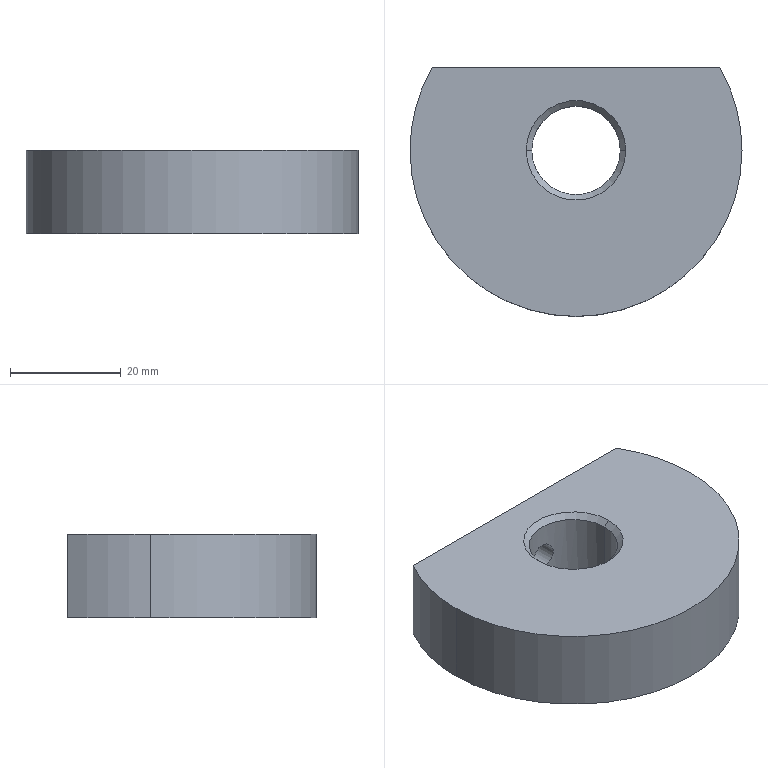Component | SolidWorks | YC1-250-09SecondDropAssembly-1_YC1-25-09-02Cam-1 | 1 solid | 14 faces | box 60 x 45 x 15 mm | volume 30912 mm3 | cylinder 7 | cone 4 | plane 3 | commonest cylinder face diameters 60 x3 5 x2 16 x2 | material Plain Carbon Steel
STEP:
#1=COLOUR_RGB('',0.7922,0.8196,0.9333);
#2=FILL_AREA_STYLE_COLOUR('',#1);
#3=FILL_AREA_STYLE('',(#2));
#4=SURFACE_STYLE_FILL_AREA(#3);
#5=SURFACE_SIDE_STYLE('',(#4));
#6=SURFACE_STYLE_USAGE(.BOTH.,#5);
#7=PRESENTATION_STYLE_ASSIGNMENT((#6));
#8=CARTESIAN_POINT('',(1.023,132.283,-41.024));
#9=VERTEX_POINT('',#8);
#10=CARTESIAN_POINT('',(1.181,131.693,-41.024));
#11=VERTEX_POINT('',#10);
#12=CARTESIAN_POINT('',(0.,131.693,-41.024));
#13=DIRECTION('',(0.,0.,-1.));
#14=DIRECTION('',(-1.,0.,0.));
#15=AXIS2_PLACEMENT_3D('',#12,#13,#14);
#16=CIRCLE('',#15,1.181);
#17=EDGE_CURVE('',#9,#11,#16,.T.);
#18=ORIENTED_EDGE('',*,*,#17,.T.);
#19=CARTESIAN_POINT('',(1.181,131.693,-41.614));
#20=VERTEX_POINT('',#19);
#21=CARTESIAN_POINT('',(1.181,131.693,-41.024));
#22=DIRECTION('',(0.,0.,-1.));
#23=VECTOR('',#22,39.37);
#24=LINE('',#21,#23);
#25=EDGE_CURVE('',#11,#20,#24,.T.);
#26=ORIENTED_EDGE('',*,*,#25,.T.);
#27=CARTESIAN_POINT('',(1.023,132.283,-41.614));
#28=VERTEX_POINT('',#27);
#29=CARTESIAN_POINT('',(0.,131.693,-41.614));
#30=DIRECTION('',(0.,0.,1.));
#31=DIRECTION('',(-1.,-0.,0.));
#32=AXIS2_PLACEMENT_3D('',#29,#30,#31);
#33=CIRCLE('',#32,1.181);
#34=EDGE_CURVE('',#20,#28,#33,.T.);
#35=ORIENTED_EDGE('',*,*,#34,.T.);
#36=CARTESIAN_POINT('',(1.023,132.283,-41.024));
#37=DIRECTION('',(0.,0.,1.));
#38=VECTOR('',#37,39.37);
#39=LINE('',#36,#38);
#40=EDGE_CURVE('',#28,#9,#39,.T.);
#41=ORIENTED_EDGE('',*,*,#40,.T.);
#42=EDGE_LOOP('',(#18,#26,#35,#41));
#43=FACE_OUTER_BOUND('',#42,.T.);
#44=CARTESIAN_POINT('',(0.,131.693,-41.024));
#45=DIRECTION('',(0.,0.,-1.));
#46=DIRECTION('',(-1.,0.,0.));
#47=AXIS2_PLACEMENT_3D('',#44,#45,#46);
#48=CYLINDRICAL_SURFACE('',#47,1.181);
#49=ADVANCED_FACE('',(#43),#48,.T.);
#50=ORIENTED_EDGE('',*,*,#25,.F.);
#51=CARTESIAN_POINT('',(-1.181,131.693,-41.024));
#52=VERTEX_POINT('',#51);
#53=CARTESIAN_POINT('',(0.,131.693,-41.024));
#54=DIRECTION('',(0.,0.,-1.));
#55=DIRECTION('',(-1.,0.,0.));
#56=AXIS2_PLACEMENT_3D('',#53,#54,#55);
#57=CIRCLE('',#56,1.181);
#58=EDGE_CURVE('',#11,#52,#57,.T.);
#59=ORIENTED_EDGE('',*,*,#58,.T.);
#60=CARTESIAN_POINT('',(-1.181,131.693,-41.614));
#61=VERTEX_POINT('',#60);
#62=CARTESIAN_POINT('',(-1.181,131.693,-41.024));
#63=DIRECTION('',(0.,0.,-1.));
#64=VECTOR('',#63,39.37);
#65=LINE('',#62,#64);
#66=EDGE_CURVE('',#52,#61,#65,.T.);
#67=ORIENTED_EDGE('',*,*,#66,.T.);
#68=CARTESIAN_POINT('',(0.,131.693,-41.614));
#69=DIRECTION('',(0.,0.,1.));
#70=DIRECTION('',(-1.,0.,0.));
#71=AXIS2_PLACEMENT_3D('',#68,#69,#70);
#72=CIRCLE('',#71,1.181);
#73=EDGE_CURVE('',#61,#20,#72,.T.);
#74=ORIENTED_EDGE('',*,*,#73,.T.);
#75=EDGE_LOOP('',(#50,#59,#67,#74));
#76=FACE_OUTER_BOUND('',#75,.T.);
#77=CARTESIAN_POINT('',(0.,131.693,-41.024));
#78=DIRECTION('',(0.,0.,-1.));
#79=DIRECTION('',(-1.,0.,0.));
#80=AXIS2_PLACEMENT_3D('',#77,#78,#79);
#81=CYLINDRICAL_SURFACE('',#80,1.181);
#82=ADVANCED_FACE('',(#76),#81,.T.);
#83=CARTESIAN_POINT('',(0.,131.378,-41.575));
#84=VERTEX_POINT('',#83);
#85=CARTESIAN_POINT('',(-0.315,131.693,-41.575));
#86=VERTEX_POINT('',#85);
#87=CARTESIAN_POINT('',(0.,131.693,-41.575));
#88=DIRECTION('',(0.,0.,-1.));
#89=DIRECTION('',(-1.,0.,0.));
#90=AXIS2_PLACEMENT_3D('',#87,#88,#89);
#91=CIRCLE('',#90,0.315);
#92=EDGE_CURVE('',#84,#86,#91,.T.);
#93=ORIENTED_EDGE('',*,*,#92,.F.);
#94=CARTESIAN_POINT('',(0.,131.339,-41.614));
#95=VERTEX_POINT('',#94);
#96=CARTESIAN_POINT('',(0.,131.339,-41.614));
#97=DIRECTION('',(0.,-0.7071,-0.7071));
#98=VECTOR('',#97,39.37);
#99=LINE('',#96,#98);
#100=EDGE_CURVE('',#84,#95,#99,.T.);
#101=ORIENTED_EDGE('',*,*,#100,.T.);
#102=CARTESIAN_POINT('',(0.,132.047,-41.614));
#103=VERTEX_POINT('',#102);
#104=CARTESIAN_POINT('',(0.,131.693,-41.614));
#105=DIRECTION('',(0.,0.,-1.));
#106=DIRECTION('',(0.,1.,0.));
#107=AXIS2_PLACEMENT_3D('',#104,#105,#106);
#108=CIRCLE('',#107,0.3543);
#109=EDGE_CURVE('',#95,#103,#108,.T.);
#110=ORIENTED_EDGE('',*,*,#109,.T.);
#111=CARTESIAN_POINT('',(0.,132.008,-41.575));
#112=VERTEX_POINT('',#111);
#113=CARTESIAN_POINT('',(0.,132.047,-41.614));
#114=DIRECTION('',(0.,0.7071,-0.7071));
#115=VECTOR('',#114,39.37);
#116=LINE('',#113,#115);
#117=EDGE_CURVE('',#112,#103,#116,.T.);
#118=ORIENTED_EDGE('',*,*,#117,.F.);
#119=CARTESIAN_POINT('',(0.,131.693,-41.575));
#120=DIRECTION('',(0.,0.,-1.));
#121=DIRECTION('',(-1.,0.,0.));
#122=AXIS2_PLACEMENT_3D('',#119,#120,#121);
#123=CIRCLE('',#122,0.315);
#124=EDGE_CURVE('',#86,#112,#123,.T.);
#125=ORIENTED_EDGE('',*,*,#124,.F.);
#126=EDGE_LOOP('',(#93,#101,#110,#118,#125));
#127=FACE_OUTER_BOUND('',#126,.T.);
#128=CARTESIAN_POINT('',(0.,131.693,-41.614));
#129=DIRECTION('',(0.,0.,-1.));
#130=DIRECTION('',(0.,1.,0.));
#131=AXIS2_PLACEMENT_3D('',#128,#129,#130);
#132=CONICAL_SURFACE('',#131,0.3543,0.7854);
#133=ADVANCED_FACE('',(#127),#132,.F.);
#134=CARTESIAN_POINT('',(0.,132.008,-41.417));
#135=VERTEX_POINT('',#134);
#136=CARTESIAN_POINT('',(0.,132.008,-41.22));
#137=VERTEX_POINT('',#136);
#138=CARTESIAN_POINT('',(0.,132.008,-41.417));
#139=CARTESIAN_POINT('',(-0.006545,132.008,-41.417));
#140=CARTESIAN_POINT('',(-0.01297,132.008,-41.417));
#141=CARTESIAN_POINT('',(-0.02561,132.007,-41.414));
#142=CARTESIAN_POINT('',(-0.03188,132.006,-41.412));
#143=CARTESIAN_POINT('',(-0.04378,132.005,-41.407));
#144=CARTESIAN_POINT('',(-0.04942,132.004,-41.404));
#145=CARTESIAN_POINT('',(-0.06008,132.002,-41.397));
#146=CARTESIAN_POINT('',(-0.0651,132.001,-41.393));
#147=CARTESIAN_POINT('',(-0.07862,131.998,-41.379));
#148=CARTESIAN_POINT('',(-0.08593,131.996,-41.369));
#149=CARTESIAN_POINT('',(-0.09332,131.994,-41.351));
#150=CARTESIAN_POINT('',(-0.09523,131.993,-41.345));
#151=CARTESIAN_POINT('',(-0.09778,131.992,-41.332));
#152=CARTESIAN_POINT('',(-0.09842,131.992,-41.325));
#153=CARTESIAN_POINT('',(-0.09843,131.992,-41.313));
#154=CARTESIAN_POINT('',(-0.09779,131.992,-41.306));
#155=CARTESIAN_POINT('',(-0.09526,131.993,-41.293));
#156=CARTESIAN_POINT('',(-0.09339,131.994,-41.287));
#157=CARTESIAN_POINT('',(-0.08843,131.995,-41.275));
#158=CARTESIAN_POINT('',(-0.08537,131.996,-41.27));
#159=CARTESIAN_POINT('',(-0.07827,131.998,-41.259));
#160=CARTESIAN_POINT('',(-0.07417,131.999,-41.254));
#161=CARTESIAN_POINT('',(-0.0651,132.001,-41.245));
#162=CARTESIAN_POINT('',(-0.06018,132.002,-41.241));
#163=CARTESIAN_POINT('',(-0.04955,132.004,-41.234));
#164=CARTESIAN_POINT('',(-0.04379,132.005,-41.231));
#165=CARTESIAN_POINT('',(-0.03194,132.006,-41.226));
#166=CARTESIAN_POINT('',(-0.0258,132.007,-41.224));
#167=CARTESIAN_POINT('',(-0.01309,132.008,-41.221));
#168=CARTESIAN_POINT('',(-0.006544,132.008,-41.22));
#169=CARTESIAN_POINT('',(0.,132.008,-41.22));
#170=B_SPLINE_CURVE_WITH_KNOTS('',3,(#138,#139,#140,#141,#142,#143,#144,#145,#146,#147,#148,#149,#150,#151,#152,#153,#154,#155,#156,#157,#158,#159,#160,#161,#162,#163,#164,#165,#166,#167,#168,#169),.UNSPECIFIED.,.F.,.F.,(4,2,2,2,2,2,2,2,2,2,2,2,2,2,2,4),(0.007863,0.008354,0.008846,0.009337,0.009828,0.01081,0.0113,0.01179,0.01229,0.01278,0.01327,0.01376,0.01425,0.01474,0.01523,0.01573),.UNSPECIFIED.);
#171=EDGE_CURVE('',#135,#137,#170,.T.);
#172=ORIENTED_EDGE('',*,*,#171,.F.);
#173=CARTESIAN_POINT('',(0.,132.283,-41.417));
#174=VERTEX_POINT('',#173);
#175=CARTESIAN_POINT('',(0.,132.283,-41.417));
#176=DIRECTION('',(0.,1.,0.));
#177=VECTOR('',#176,39.37);
#178=LINE('',#175,#177);
#179=EDGE_CURVE('',#135,#174,#178,.T.);
#180=ORIENTED_EDGE('',*,*,#179,.T.);
#181=CARTESIAN_POINT('',(0.,132.283,-41.22));
#182=VERTEX_POINT('',#181);
#183=CARTESIAN_POINT('',(0.,132.283,-41.319));
#184=DIRECTION('',(0.,1.,0.));
#185=DIRECTION('',(0.,0.,1.));
#186=AXIS2_PLACEMENT_3D('',#183,#184,#185);
#187=CIRCLE('',#186,0.09843);
#188=EDGE_CURVE('',#174,#182,#187,.T.);
#189=ORIENTED_EDGE('',*,*,#188,.T.);
#190=CARTESIAN_POINT('',(0.,132.283,-41.22));
#191=DIRECTION('',(0.,1.,0.));
#192=VECTOR('',#191,39.37);
#193=LINE('',#190,#192);
#194=EDGE_CURVE('',#137,#182,#193,.T.);
#195=ORIENTED_EDGE('',*,*,#194,.F.);
#196=EDGE_LOOP('',(#172,#180,#189,#195));
#197=FACE_OUTER_BOUND('',#196,.T.);
#198=CARTESIAN_POINT('',(0.,132.283,-41.319));
#199=DIRECTION('',(0.,1.,0.));
#200=DIRECTION('',(0.,0.,1.));
#201=AXIS2_PLACEMENT_3D('',#198,#199,#200);
#202=CYLINDRICAL_SURFACE('',#201,0.09843);
#203=ADVANCED_FACE('',(#197),#202,.F.);
#204=CARTESIAN_POINT('',(0.315,131.693,-41.063));
#205=VERTEX_POINT('',#204);
#206=CARTESIAN_POINT('',(-0.315,131.693,-41.063));
#207=VERTEX_POINT('',#206);
#208=CARTESIAN_POINT('',(0.,131.693,-41.063));
#209=DIRECTION('',(0.,0.,-1.));
#210=DIRECTION('',(-1.,0.,0.));
#211=AXIS2_PLACEMENT_3D('',#208,#209,#210);
#212=CIRCLE('',#211,0.315);
#213=EDGE_CURVE('',#205,#207,#212,.T.);
#214=ORIENTED_EDGE('',*,*,#213,.F.);
#215=CARTESIAN_POINT('',(0.315,131.693,-41.575));
#216=VERTEX_POINT('',#215);
#217=CARTESIAN_POINT('',(0.315,131.693,-41.024));
#218=DIRECTION('',(0.,0.,-1.));
#219=VECTOR('',#218,39.37);
#220=LINE('',#217,#219);
#221=EDGE_CURVE('',#205,#216,#220,.T.);
#222=ORIENTED_EDGE('',*,*,#221,.T.);
#223=CARTESIAN_POINT('',(0.,131.693,-41.575));
#224=DIRECTION('',(0.,0.,-1.));
#225=DIRECTION('',(-1.,0.,0.));
#226=AXIS2_PLACEMENT_3D('',#223,#224,#225);
#227=CIRCLE('',#226,0.315);
#228=EDGE_CURVE('',#216,#84,#227,.T.);
#229=ORIENTED_EDGE('',*,*,#228,.T.);
#230=ORIENTED_EDGE('',*,*,#92,.T.);
#231=CARTESIAN_POINT('',(-0.315,131.693,-41.024));
#232=DIRECTION('',(0.,0.,-1.));
#233=VECTOR('',#232,39.37);
#234=LINE('',#231,#233);
#235=EDGE_CURVE('',#207,#86,#234,.T.);
#236=ORIENTED_EDGE('',*,*,#235,.F.);
#237=EDGE_LOOP('',(#214,#222,#229,#230,#236));
#238=FACE_OUTER_BOUND('',#237,.T.);
#239=CARTESIAN_POINT('',(0.,131.693,-41.024));
#240=DIRECTION('',(0.,0.,-1.));
#241=DIRECTION('',(-1.,0.,0.));
#242=AXIS2_PLACEMENT_3D('',#239,#240,#241);
#243=CYLINDRICAL_SURFACE('',#242,0.315);
#244=ADVANCED_FACE('',(#238),#243,.F.);
#245=ORIENTED_EDGE('',*,*,#213,.T.);
#246=CARTESIAN_POINT('',(-0.3543,131.693,-41.024));
#247=VERTEX_POINT('',#246);
#248=CARTESIAN_POINT('',(-0.3543,131.693,-41.024));
#249=DIRECTION('',(-0.7071,0.,0.7071));
#250=VECTOR('',#249,39.37);
#251=LINE('',#248,#250);
#252=EDGE_CURVE('',#207,#247,#251,.T.);
#253=ORIENTED_EDGE('',*,*,#252,.T.);
#254=CARTESIAN_POINT('',(0.3543,131.693,-41.024));
#255=VERTEX_POINT('',#254);
#256=CARTESIAN_POINT('',(0.,131.693,-41.024));
#257=DIRECTION('',(0.,0.,-1.));
#258=DIRECTION('',(1.,0.,0.));
#259=AXIS2_PLACEMENT_3D('',#256,#257,#258);
#260=CIRCLE('',#259,0.3543);
#261=EDGE_CURVE('',#255,#247,#260,.T.);
#262=ORIENTED_EDGE('',*,*,#261,.F.);
#263=CARTESIAN_POINT('',(0.3543,131.693,-41.024));
#264=DIRECTION('',(0.7071,0.,0.7071));
#265=VECTOR('',#264,39.37);
#266=LINE('',#263,#265);
#267=EDGE_CURVE('',#205,#255,#266,.T.);
#268=ORIENTED_EDGE('',*,*,#267,.F.);
#269=EDGE_LOOP('',(#245,#253,#262,#268));
#270=FACE_OUTER_BOUND('',#269,.T.);
#271=CARTESIAN_POINT('',(0.,131.693,-41.024));
#272=DIRECTION('',(0.,0.,1.));
#273=DIRECTION('',(1.,0.,0.));
#274=AXIS2_PLACEMENT_3D('',#271,#272,#273);
#275=CONICAL_SURFACE('',#274,0.3543,0.7854);
#276=ADVANCED_FACE('',(#270),#275,.F.);
#277=CARTESIAN_POINT('',(-1.023,132.283,-41.614));
#278=VERTEX_POINT('',#277);
#279=CARTESIAN_POINT('',(0.,132.283,-41.614));
#280=DIRECTION('',(-1.,0.,0.));
#281=VECTOR('',#280,39.37);
#282=LINE('',#279,#281);
#283=EDGE_CURVE('',#28,#278,#282,.T.);
#284=ORIENTED_EDGE('',*,*,#283,.F.);
#285=ORIENTED_EDGE('',*,*,#34,.F.);
#286=ORIENTED_EDGE('',*,*,#73,.F.);
#287=CARTESIAN_POINT('',(0.,131.693,-41.614));
#288=DIRECTION('',(0.,0.,1.));
#289=DIRECTION('',(-1.,-0.,0.));
#290=AXIS2_PLACEMENT_3D('',#287,#288,#289);
#291=CIRCLE('',#290,1.181);
#292=EDGE_CURVE('',#278,#61,#291,.T.);
#293=ORIENTED_EDGE('',*,*,#292,.F.);
#294=EDGE_LOOP('',(#284,#285,#286,#293));
#295=FACE_OUTER_BOUND('',#294,.T.);
#296=CARTESIAN_POINT('',(0.,131.693,-41.614));
#297=DIRECTION('',(0.,0.,-1.));
#298=DIRECTION('',(0.,1.,0.));
#299=AXIS2_PLACEMENT_3D('',#296,#297,#298);
#300=CIRCLE('',#299,0.3543);
#301=EDGE_CURVE('',#103,#95,#300,.T.);
#302=ORIENTED_EDGE('',*,*,#301,.F.);
#303=ORIENTED_EDGE('',*,*,#109,.F.);
#304=EDGE_LOOP('',(#302,#303));
#305=FACE_BOUND('',#304,.T.);
#306=CARTESIAN_POINT('',(0.,131.693,-41.614));
#307=DIRECTION('',(0.,0.,1.));
#308=DIRECTION('',(1.,0.,0.));
#309=AXIS2_PLACEMENT_3D('',#306,#307,#308);
#310=PLANE('',#309);
#311=ADVANCED_FACE('',(#295,#305),#310,.F.);
#312=ORIENTED_EDGE('',*,*,#66,.F.);
#313=CARTESIAN_POINT('',(-1.023,132.283,-41.024));
#314=VERTEX_POINT('',#313);
#315=CARTESIAN_POINT('',(0.,131.693,-41.024));
#316=DIRECTION('',(0.,0.,-1.));
#317=DIRECTION('',(-1.,0.,0.));
#318=AXIS2_PLACEMENT_3D('',#315,#316,#317);
#319=CIRCLE('',#318,1.181);
#320=EDGE_CURVE('',#52,#314,#319,.T.);
#321=ORIENTED_EDGE('',*,*,#320,.T.);
#322=CARTESIAN_POINT('',(-1.023,132.283,-41.024));
#323=DIRECTION('',(0.,0.,-1.));
#324=VECTOR('',#323,39.37);
#325=LINE('',#322,#324);
#326=EDGE_CURVE('',#314,#278,#325,.T.);
#327=ORIENTED_EDGE('',*,*,#326,.T.);
#328=ORIENTED_EDGE('',*,*,#292,.T.);
#329=EDGE_LOOP('',(#312,#321,#327,#328));
#330=FACE_OUTER_BOUND('',#329,.T.);
#331=CARTESIAN_POINT('',(0.,131.693,-41.024));
#332=DIRECTION('',(0.,0.,-1.));
#333=DIRECTION('',(-1.,0.,0.));
#334=AXIS2_PLACEMENT_3D('',#331,#332,#333);
#335=CYLINDRICAL_SURFACE('',#334,1.181);
#336=ADVANCED_FACE('',(#330),#335,.T.);
#337=CARTESIAN_POINT('',(0.,132.283,-41.319));
#338=DIRECTION('',(0.,1.,0.));
#339=DIRECTION('',(0.,0.,1.));
#340=AXIS2_PLACEMENT_3D('',#337,#338,#339);
#341=CIRCLE('',#340,0.09843);
#342=EDGE_CURVE('',#182,#174,#341,.T.);
#343=ORIENTED_EDGE('',*,*,#342,.F.);
#344=ORIENTED_EDGE('',*,*,#188,.F.);
#345=EDGE_LOOP('',(#343,#344));
#346=FACE_BOUND('',#345,.T.);
#347=ORIENTED_EDGE('',*,*,#326,.F.);
#348=CARTESIAN_POINT('',(-1.023,132.283,-41.024));
#349=DIRECTION('',(-1.,0.,0.));
#350=VECTOR('',#349,39.37);
#351=LINE('',#348,#350);
#352=EDGE_CURVE('',#9,#314,#351,.T.);
#353=ORIENTED_EDGE('',*,*,#352,.F.);
#354=ORIENTED_EDGE('',*,*,#40,.F.);
#355=ORIENTED_EDGE('',*,*,#283,.T.);
#356=EDGE_LOOP('',(#347,#353,#354,#355));
#357=FACE_OUTER_BOUND('',#356,.T.);
#358=CARTESIAN_POINT('',(-1.023,132.283,-41.024));
#359=DIRECTION('',(0.,-1.,0.));
#360=DIRECTION('',(0.,0.,-1.));
#361=AXIS2_PLACEMENT_3D('',#358,#359,#360);
#362=PLANE('',#361);
#363=ADVANCED_FACE('',(#346,#357),#362,.F.);
#364=ORIENTED_EDGE('',*,*,#100,.F.);
#365=ORIENTED_EDGE('',*,*,#228,.F.);
#366=CARTESIAN_POINT('',(0.,131.693,-41.575));
#367=DIRECTION('',(0.,0.,-1.));
#368=DIRECTION('',(-1.,0.,0.));
#369=AXIS2_PLACEMENT_3D('',#366,#367,#368);
#370=CIRCLE('',#369,0.315);
#371=EDGE_CURVE('',#112,#216,#370,.T.);
#372=ORIENTED_EDGE('',*,*,#371,.F.);
#373=ORIENTED_EDGE('',*,*,#117,.T.);
#374=ORIENTED_EDGE('',*,*,#301,.T.);
#375=EDGE_LOOP('',(#364,#365,#372,#373,#374));
#376=FACE_OUTER_BOUND('',#375,.T.);
#377=CARTESIAN_POINT('',(0.,131.693,-41.614));
#378=DIRECTION('',(0.,0.,-1.));
#379=DIRECTION('',(0.,1.,0.));
#380=AXIS2_PLACEMENT_3D('',#377,#378,#379);
#381=CONICAL_SURFACE('',#380,0.3543,0.7854);
#382=ADVANCED_FACE('',(#376),#381,.F.);
#383=ORIENTED_EDGE('',*,*,#17,.F.);
#384=ORIENTED_EDGE('',*,*,#352,.T.);
#385=ORIENTED_EDGE('',*,*,#320,.F.);
#386=ORIENTED_EDGE('',*,*,#58,.F.);
#387=EDGE_LOOP('',(#383,#384,#385,#386));
#388=FACE_OUTER_BOUND('',#387,.T.);
#389=ORIENTED_EDGE('',*,*,#261,.T.);
#390=CARTESIAN_POINT('',(0.,131.693,-41.024));
#391=DIRECTION('',(0.,0.,-1.));
#392=DIRECTION('',(1.,0.,0.));
#393=AXIS2_PLACEMENT_3D('',#390,#391,#392);
#394=CIRCLE('',#393,0.3543);
#395=EDGE_CURVE('',#247,#255,#394,.T.);
#396=ORIENTED_EDGE('',*,*,#395,.T.);
#397=EDGE_LOOP('',(#389,#396));
#398=FACE_BOUND('',#397,.T.);
#399=CARTESIAN_POINT('',(0.,131.693,-41.024));
#400=DIRECTION('',(0.,0.,1.));
#401=DIRECTION('',(1.,0.,0.));
#402=AXIS2_PLACEMENT_3D('',#399,#400,#401);
#403=PLANE('',#402);
#404=ADVANCED_FACE('',(#388,#398),#403,.T.);
#405=ORIENTED_EDGE('',*,*,#179,.F.);
#406=CARTESIAN_POINT('',(0.,132.008,-41.22));
#407=CARTESIAN_POINT('',(0.006545,132.008,-41.22));
#408=CARTESIAN_POINT('',(0.01297,132.008,-41.221));
#409=CARTESIAN_POINT('',(0.02561,132.007,-41.224));
#410=CARTESIAN_POINT('',(0.03188,132.006,-41.226));
#411=CARTESIAN_POINT('',(0.04378,132.005,-41.231));
#412=CARTESIAN_POINT('',(0.04942,132.004,-41.234));
#413=CARTESIAN_POINT('',(0.06008,132.002,-41.241));
#414=CARTESIAN_POINT('',(0.0651,132.001,-41.245));
#415=CARTESIAN_POINT('',(0.07862,131.998,-41.258));
#416=CARTESIAN_POINT('',(0.08593,131.996,-41.269));
#417=CARTESIAN_POINT('',(0.09332,131.994,-41.287));
#418=CARTESIAN_POINT('',(0.09523,131.993,-41.293));
#419=CARTESIAN_POINT('',(0.09778,131.992,-41.306));
#420=CARTESIAN_POINT('',(0.09842,131.992,-41.312));
#421=CARTESIAN_POINT('',(0.09843,131.992,-41.325));
#422=CARTESIAN_POINT('',(0.09779,131.992,-41.332));
#423=CARTESIAN_POINT('',(0.09526,131.993,-41.344));
#424=CARTESIAN_POINT('',(0.09339,131.994,-41.351));
#425=CARTESIAN_POINT('',(0.08843,131.995,-41.363));
#426=CARTESIAN_POINT('',(0.08537,131.996,-41.368));
#427=CARTESIAN_POINT('',(0.07827,131.998,-41.379));
#428=CARTESIAN_POINT('',(0.07417,131.999,-41.384));
#429=CARTESIAN_POINT('',(0.0651,132.001,-41.393));
#430=CARTESIAN_POINT('',(0.06018,132.002,-41.397));
#431=CARTESIAN_POINT('',(0.04955,132.004,-41.404));
#432=CARTESIAN_POINT('',(0.04379,132.005,-41.407));
#433=CARTESIAN_POINT('',(0.03194,132.006,-41.412));
#434=CARTESIAN_POINT('',(0.0258,132.007,-41.414));
#435=CARTESIAN_POINT('',(0.01309,132.008,-41.417));
#436=CARTESIAN_POINT('',(0.006546,132.008,-41.417));
#437=CARTESIAN_POINT('',(0.,132.008,-41.417));
#438=B_SPLINE_CURVE_WITH_KNOTS('',3,(#406,#407,#408,#409,#410,#411,#412,#413,#414,#415,#416,#417,#418,#419,#420,#421,#422,#423,#424,#425,#426,#427,#428,#429,#430,#431,#432,#433,#434,#435,#436,#437),.UNSPECIFIED.,.F.,.F.,(4,2,2,2,2,2,2,2,2,2,2,2,2,2,2,4),(0.,0.0004914,0.0009829,0.001474,0.001966,0.002949,0.00344,0.003931,0.004423,0.004914,0.005406,0.005897,0.006389,0.00688,0.007371,0.007863),.UNSPECIFIED.);
#439=EDGE_CURVE('',#137,#135,#438,.T.);
#440=ORIENTED_EDGE('',*,*,#439,.F.);
#441=ORIENTED_EDGE('',*,*,#194,.T.);
#442=ORIENTED_EDGE('',*,*,#342,.T.);
#443=EDGE_LOOP('',(#405,#440,#441,#442));
#444=FACE_OUTER_BOUND('',#443,.T.);
#445=CARTESIAN_POINT('',(0.,132.283,-41.319));
#446=DIRECTION('',(0.,1.,0.));
#447=DIRECTION('',(0.,0.,1.));
#448=AXIS2_PLACEMENT_3D('',#445,#446,#447);
#449=CYLINDRICAL_SURFACE('',#448,0.09843);
#450=ADVANCED_FACE('',(#444),#449,.F.);
#451=ORIENTED_EDGE('',*,*,#221,.F.);
#452=CARTESIAN_POINT('',(0.,131.693,-41.063));
#453=DIRECTION('',(0.,0.,-1.));
#454=DIRECTION('',(-1.,0.,0.));
#455=AXIS2_PLACEMENT_3D('',#452,#453,#454);
#456=CIRCLE('',#455,0.315);
#457=EDGE_CURVE('',#207,#205,#456,.T.);
#458=ORIENTED_EDGE('',*,*,#457,.F.);
#459=ORIENTED_EDGE('',*,*,#235,.T.);
#460=ORIENTED_EDGE('',*,*,#124,.T.);
#461=ORIENTED_EDGE('',*,*,#371,.T.);
#462=EDGE_LOOP('',(#451,#458,#459,#460,#461));
#463=FACE_OUTER_BOUND('',#462,.T.);
#464=ORIENTED_EDGE('',*,*,#439,.T.);
#465=ORIENTED_EDGE('',*,*,#171,.T.);
#466=EDGE_LOOP('',(#464,#465));
#467=FACE_BOUND('',#466,.T.);
#468=CARTESIAN_POINT('',(0.,131.693,-41.024));
#469=DIRECTION('',(0.,0.,-1.));
#470=DIRECTION('',(-1.,0.,0.));
#471=AXIS2_PLACEMENT_3D('',#468,#469,#470);
#472=CYLINDRICAL_SURFACE('',#471,0.315);
#473=ADVANCED_FACE('',(#463,#467),#472,.F.);
#474=ORIENTED_EDGE('',*,*,#252,.F.);
#475=ORIENTED_EDGE('',*,*,#457,.T.);
#476=ORIENTED_EDGE('',*,*,#267,.T.);
#477=ORIENTED_EDGE('',*,*,#395,.F.);
#478=EDGE_LOOP('',(#474,#475,#476,#477));
#479=FACE_OUTER_BOUND('',#478,.T.);
#480=CARTESIAN_POINT('',(0.,131.693,-41.024));
#481=DIRECTION('',(0.,0.,1.));
#482=DIRECTION('',(1.,0.,0.));
#483=AXIS2_PLACEMENT_3D('',#480,#481,#482);
#484=CONICAL_SURFACE('',#483,0.3543,0.7854);
#485=ADVANCED_FACE('',(#479),#484,.F.);
#486=CLOSED_SHELL('',(#49,#82,#133,#203,#244,#276,#311,#336,#363,#382,#404,#450,#473,#485));
#487=MANIFOLD_SOLID_BREP('',#486);
#488=STYLED_ITEM('',(#7),#487);
#489=PRESENTATION_LAYER_ASSIGNMENT('','',(#488));
#490=CARTESIAN_POINT('',(0.,0.,0.));
#491=DIRECTION('',(0.,0.,1.));
#492=DIRECTION('',(1.,0.,0.));
#493=AXIS2_PLACEMENT_3D('',#490,#491,#492);
#494=(LENGTH_UNIT()NAMED_UNIT(*)SI_UNIT($,.METRE.));
#495=LENGTH_MEASURE_WITH_UNIT(LENGTH_MEASURE(0.0254),#494);
#496=DIMENSIONAL_EXPONENTS(1.,0.,0.,0.,0.,0.,0.);
#497=(CONVERSION_BASED_UNIT('',#495)LENGTH_UNIT()NAMED_UNIT(#496));
#498=UNCERTAINTY_MEASURE_WITH_UNIT(LENGTH_MEASURE(0.00001),#497,'','');
#499=(NAMED_UNIT(*)PLANE_ANGLE_UNIT()SI_UNIT($,.RADIAN.));
#500=(NAMED_UNIT(*)SI_UNIT($,.STERADIAN.)SOLID_ANGLE_UNIT());
#501=(GEOMETRIC_REPRESENTATION_CONTEXT(3)GLOBAL_UNCERTAINTY_ASSIGNED_CONTEXT((#498))GLOBAL_UNIT_ASSIGNED_CONTEXT((#497,#499,#500))REPRESENTATION_CONTEXT('',''));
#502=ADVANCED_BREP_SHAPE_REPRESENTATION('',(#487,#493),#501);
#503=(LENGTH_UNIT()NAMED_UNIT(*)SI_UNIT($,.METRE.));
#504=LENGTH_MEASURE_WITH_UNIT(LENGTH_MEASURE(0.0254),#503);
#505=DIMENSIONAL_EXPONENTS(1.,0.,0.,0.,0.,0.,0.);
#506=(CONVERSION_BASED_UNIT('',#504)LENGTH_UNIT()NAMED_UNIT(#505));
#507=UNCERTAINTY_MEASURE_WITH_UNIT(LENGTH_MEASURE(0.00001),#506,'','');
#508=(NAMED_UNIT(*)PLANE_ANGLE_UNIT()SI_UNIT($,.RADIAN.));
#509=(NAMED_UNIT(*)SI_UNIT($,.STERADIAN.)SOLID_ANGLE_UNIT());
#510=(GEOMETRIC_REPRESENTATION_CONTEXT(3)GLOBAL_UNCERTAINTY_ASSIGNED_CONTEXT((#507))GLOBAL_UNIT_ASSIGNED_CONTEXT((#506,#508,#509))REPRESENTATION_CONTEXT('',''));
#511=MECHANICAL_DESIGN_GEOMETRIC_PRESENTATION_REPRESENTATION('',(#488),#510);